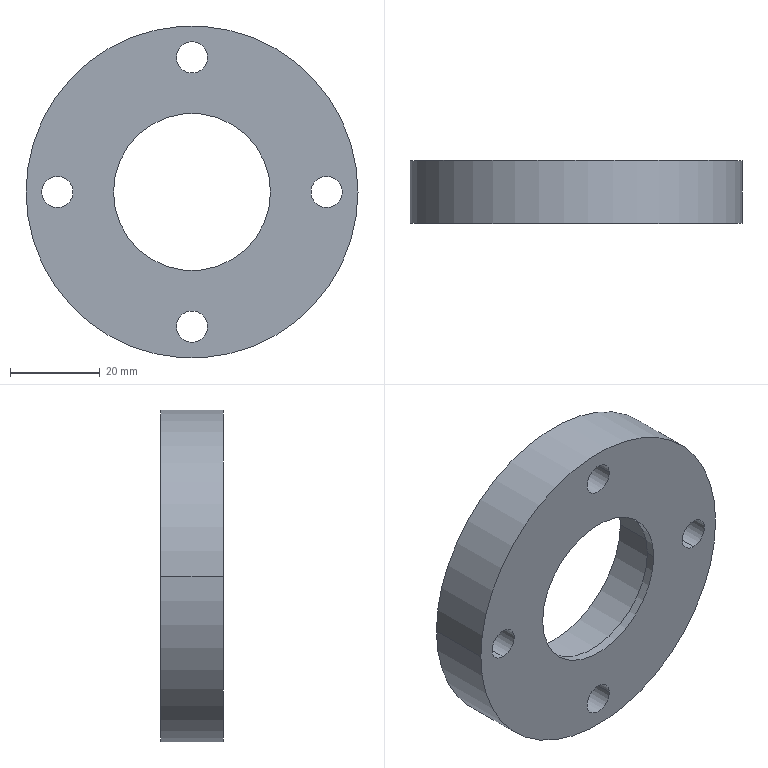Component | SolidWorks | -6004BearingHousing-1 | 1 solid | 29 faces | box 74 x 14 x 74 mm | volume 38150 mm3 | cylinder 22 | plane 7 | commonest cylinder face diameters 11 x8 7 x8 74 x2 42 x2 35 x2
build123d program:
from build123d import *

# Parameters (mm, degrees)
CYLINDRICAL_COUNTERSUNK_HOLE_FOR_M6_HEX_D           = 7
CYLINDRICAL_COUNTERSUNK_HOLE_FOR_M6_HEX_CBORE_D     = 11
CYLINDRICAL_COUNTERSUNK_HOLE_FOR_M6_HEX_CBORE_DEPTH = 6
CIRPATTERN1_COUNT                                   = 4


with BuildPart() as part:
    # Sketch1 → Revolve1 (revolve)
    with BuildSketch(Plane.XY):
        Polygon((17.5, 0), (17.5, 2), (21, 2), (21, 14), (37, 14), (37, 0), align=None)
    revolve(axis=Axis((0, -515.921, 0), (0, 1, 0)))

    # Cylindrical Countersunk Hole for M6 Hex (through all)
    with Locations(Plane(origin=(0, 14, 0), x_dir=(1, 0, 0), z_dir=(0, 1, 0))):
        with Locations((-30, 0)):
            cylindrical_countersunk_hole_for_m6_hex = CounterBoreHole(CYLINDRICAL_COUNTERSUNK_HOLE_FOR_M6_HEX_D / 2, CYLINDRICAL_COUNTERSUNK_HOLE_FOR_M6_HEX_CBORE_D / 2, CYLINDRICAL_COUNTERSUNK_HOLE_FOR_M6_HEX_CBORE_DEPTH)

    # CirPattern1: Cylindrical Countersunk Hole for M6 Hex ×4 about axis
    cirpattern1_axis = Axis((0, 0, 0), (0, 1, 0))
    for i in range(1, CIRPATTERN1_COUNT):
        add(cylindrical_countersunk_hole_for_m6_hex.rotate(cirpattern1_axis, i * 360 / CIRPATTERN1_COUNT), mode=Mode.SUBTRACT)


solid = part.part

# Placed as in the assembly
solid = solid.moved(Location((205, 1451, -173), (0, 0, 0)))
STEP:
#1=CARTESIAN_POINT('',(7.854,57.441,-5.63));
#2=VERTEX_POINT('',#1);
#3=CARTESIAN_POINT('',(8.287,57.441,-5.63));
#4=VERTEX_POINT('',#3);
#5=CARTESIAN_POINT('',(8.071,57.441,-5.63));
#6=DIRECTION('',(-0.,1.,-0.));
#7=DIRECTION('',(1.,0.,0.));
#8=AXIS2_PLACEMENT_3D('',#5,#6,#7);
#9=CIRCLE('',#8,0.2165);
#10=EDGE_CURVE('',#2,#4,#9,.T.);
#11=ORIENTED_EDGE('',*,*,#10,.F.);
#12=CARTESIAN_POINT('',(7.854,57.677,-5.63));
#13=VERTEX_POINT('',#12);
#14=CARTESIAN_POINT('',(7.854,57.677,-5.63));
#15=DIRECTION('',(-0.,1.,-0.));
#16=VECTOR('',#15,39.37);
#17=LINE('',#14,#16);
#18=EDGE_CURVE('',#2,#13,#17,.T.);
#19=ORIENTED_EDGE('',*,*,#18,.T.);
#20=CARTESIAN_POINT('',(8.287,57.677,-5.63));
#21=VERTEX_POINT('',#20);
#22=CARTESIAN_POINT('',(8.071,57.677,-5.63));
#23=DIRECTION('',(-0.,1.,-0.));
#24=DIRECTION('',(1.,0.,0.));
#25=AXIS2_PLACEMENT_3D('',#22,#23,#24);
#26=CIRCLE('',#25,0.2165);
#27=EDGE_CURVE('',#13,#21,#26,.T.);
#28=ORIENTED_EDGE('',*,*,#27,.T.);
#29=CARTESIAN_POINT('',(8.287,57.677,-5.63));
#30=DIRECTION('',(-0.,1.,-0.));
#31=VECTOR('',#30,39.37);
#32=LINE('',#29,#31);
#33=EDGE_CURVE('',#4,#21,#32,.T.);
#34=ORIENTED_EDGE('',*,*,#33,.F.);
#35=EDGE_LOOP('',(#11,#19,#28,#34));
#36=FACE_OUTER_BOUND('',#35,.T.);
#37=CARTESIAN_POINT('',(8.071,57.677,-5.63));
#38=DIRECTION('',(-0.,1.,-0.));
#39=DIRECTION('',(1.,0.,0.));
#40=AXIS2_PLACEMENT_3D('',#37,#38,#39);
#41=CYLINDRICAL_SURFACE('',#40,0.2165);
#42=ADVANCED_FACE('',(#36),#41,.F.);
#43=CARTESIAN_POINT('',(7.933,57.126,-5.63));
#44=VERTEX_POINT('',#43);
#45=CARTESIAN_POINT('',(8.209,57.126,-5.63));
#46=VERTEX_POINT('',#45);
#47=CARTESIAN_POINT('',(8.071,57.126,-5.63));
#48=DIRECTION('',(-0.,1.,-0.));
#49=DIRECTION('',(1.,0.,0.));
#50=AXIS2_PLACEMENT_3D('',#47,#48,#49);
#51=CIRCLE('',#50,0.1378);
#52=EDGE_CURVE('',#44,#46,#51,.T.);
#53=ORIENTED_EDGE('',*,*,#52,.F.);
#54=CARTESIAN_POINT('',(7.933,57.441,-5.63));
#55=VERTEX_POINT('',#54);
#56=CARTESIAN_POINT('',(7.933,57.677,-5.63));
#57=DIRECTION('',(-0.,1.,-0.));
#58=VECTOR('',#57,39.37);
#59=LINE('',#56,#58);
#60=EDGE_CURVE('',#44,#55,#59,.T.);
#61=ORIENTED_EDGE('',*,*,#60,.T.);
#62=CARTESIAN_POINT('',(8.209,57.441,-5.63));
#63=VERTEX_POINT('',#62);
#64=CARTESIAN_POINT('',(8.071,57.441,-5.63));
#65=DIRECTION('',(-0.,1.,-0.));
#66=DIRECTION('',(1.,0.,0.));
#67=AXIS2_PLACEMENT_3D('',#64,#65,#66);
#68=CIRCLE('',#67,0.1378);
#69=EDGE_CURVE('',#55,#63,#68,.T.);
#70=ORIENTED_EDGE('',*,*,#69,.T.);
#71=CARTESIAN_POINT('',(8.209,57.677,-5.63));
#72=DIRECTION('',(-0.,1.,-0.));
#73=VECTOR('',#72,39.37);
#74=LINE('',#71,#73);
#75=EDGE_CURVE('',#46,#63,#74,.T.);
#76=ORIENTED_EDGE('',*,*,#75,.F.);
#77=EDGE_LOOP('',(#53,#61,#70,#76));
#78=FACE_OUTER_BOUND('',#77,.T.);
#79=CARTESIAN_POINT('',(8.071,57.677,-5.63));
#80=DIRECTION('',(-0.,1.,-0.));
#81=DIRECTION('',(1.,0.,0.));
#82=AXIS2_PLACEMENT_3D('',#79,#80,#81);
#83=CYLINDRICAL_SURFACE('',#82,0.1378);
#84=ADVANCED_FACE('',(#78),#83,.F.);
#85=CARTESIAN_POINT('',(9.252,57.441,-6.594));
#86=VERTEX_POINT('',#85);
#87=CARTESIAN_POINT('',(9.252,57.441,-7.028));
#88=VERTEX_POINT('',#87);
#89=CARTESIAN_POINT('',(9.252,57.441,-6.811));
#90=DIRECTION('',(-0.,1.,0.));
#91=DIRECTION('',(0.,0.,-1.));
#92=AXIS2_PLACEMENT_3D('',#89,#90,#91);
#93=CIRCLE('',#92,0.2165);
#94=EDGE_CURVE('',#86,#88,#93,.T.);
#95=ORIENTED_EDGE('',*,*,#94,.F.);
#96=CARTESIAN_POINT('',(9.252,57.677,-6.594));
#97=VERTEX_POINT('',#96);
#98=CARTESIAN_POINT('',(9.252,57.677,-6.594));
#99=DIRECTION('',(-0.,1.,0.));
#100=VECTOR('',#99,39.37);
#101=LINE('',#98,#100);
#102=EDGE_CURVE('',#86,#97,#101,.T.);
#103=ORIENTED_EDGE('',*,*,#102,.T.);
#104=CARTESIAN_POINT('',(9.252,57.677,-7.028));
#105=VERTEX_POINT('',#104);
#106=CARTESIAN_POINT('',(9.252,57.677,-6.811));
#107=DIRECTION('',(-0.,1.,0.));
#108=DIRECTION('',(0.,0.,-1.));
#109=AXIS2_PLACEMENT_3D('',#106,#107,#108);
#110=CIRCLE('',#109,0.2165);
#111=EDGE_CURVE('',#97,#105,#110,.T.);
#112=ORIENTED_EDGE('',*,*,#111,.T.);
#113=CARTESIAN_POINT('',(9.252,57.677,-7.028));
#114=DIRECTION('',(-0.,1.,0.));
#115=VECTOR('',#114,39.37);
#116=LINE('',#113,#115);
#117=EDGE_CURVE('',#88,#105,#116,.T.);
#118=ORIENTED_EDGE('',*,*,#117,.F.);
#119=EDGE_LOOP('',(#95,#103,#112,#118));
#120=FACE_OUTER_BOUND('',#119,.T.);
#121=CARTESIAN_POINT('',(9.252,57.677,-6.811));
#122=DIRECTION('',(-0.,1.,0.));
#123=DIRECTION('',(0.,0.,-1.));
#124=AXIS2_PLACEMENT_3D('',#121,#122,#123);
#125=CYLINDRICAL_SURFACE('',#124,0.2165);
#126=ADVANCED_FACE('',(#120),#125,.F.);
#127=CARTESIAN_POINT('',(9.252,57.126,-6.673));
#128=VERTEX_POINT('',#127);
#129=CARTESIAN_POINT('',(9.252,57.126,-6.949));
#130=VERTEX_POINT('',#129);
#131=CARTESIAN_POINT('',(9.252,57.126,-6.811));
#132=DIRECTION('',(-0.,1.,0.));
#133=DIRECTION('',(0.,0.,-1.));
#134=AXIS2_PLACEMENT_3D('',#131,#132,#133);
#135=CIRCLE('',#134,0.1378);
#136=EDGE_CURVE('',#128,#130,#135,.T.);
#137=ORIENTED_EDGE('',*,*,#136,.F.);
#138=CARTESIAN_POINT('',(9.252,57.441,-6.673));
#139=VERTEX_POINT('',#138);
#140=CARTESIAN_POINT('',(9.252,57.677,-6.673));
#141=DIRECTION('',(-0.,1.,0.));
#142=VECTOR('',#141,39.37);
#143=LINE('',#140,#142);
#144=EDGE_CURVE('',#128,#139,#143,.T.);
#145=ORIENTED_EDGE('',*,*,#144,.T.);
#146=CARTESIAN_POINT('',(9.252,57.441,-6.949));
#147=VERTEX_POINT('',#146);
#148=CARTESIAN_POINT('',(9.252,57.441,-6.811));
#149=DIRECTION('',(-0.,1.,0.));
#150=DIRECTION('',(0.,0.,-1.));
#151=AXIS2_PLACEMENT_3D('',#148,#149,#150);
#152=CIRCLE('',#151,0.1378);
#153=EDGE_CURVE('',#139,#147,#152,.T.);
#154=ORIENTED_EDGE('',*,*,#153,.T.);
#155=CARTESIAN_POINT('',(9.252,57.677,-6.949));
#156=DIRECTION('',(-0.,1.,0.));
#157=VECTOR('',#156,39.37);
#158=LINE('',#155,#157);
#159=EDGE_CURVE('',#130,#147,#158,.T.);
#160=ORIENTED_EDGE('',*,*,#159,.F.);
#161=EDGE_LOOP('',(#137,#145,#154,#160));
#162=FACE_OUTER_BOUND('',#161,.T.);
#163=CARTESIAN_POINT('',(9.252,57.677,-6.811));
#164=DIRECTION('',(-0.,1.,0.));
#165=DIRECTION('',(0.,0.,-1.));
#166=AXIS2_PLACEMENT_3D('',#163,#164,#165);
#167=CYLINDRICAL_SURFACE('',#166,0.1378);
#168=ADVANCED_FACE('',(#162),#167,.F.);
#169=CARTESIAN_POINT('',(8.287,57.441,-7.992));
#170=VERTEX_POINT('',#169);
#171=CARTESIAN_POINT('',(7.854,57.441,-7.992));
#172=VERTEX_POINT('',#171);
#173=CARTESIAN_POINT('',(8.071,57.441,-7.992));
#174=DIRECTION('',(-0.,1.,0.));
#175=DIRECTION('',(-1.,0.,-0.));
#176=AXIS2_PLACEMENT_3D('',#173,#174,#175);
#177=CIRCLE('',#176,0.2165);
#178=EDGE_CURVE('',#170,#172,#177,.T.);
#179=ORIENTED_EDGE('',*,*,#178,.F.);
#180=CARTESIAN_POINT('',(8.287,57.677,-7.992));
#181=VERTEX_POINT('',#180);
#182=CARTESIAN_POINT('',(8.287,57.677,-7.992));
#183=DIRECTION('',(-0.,1.,0.));
#184=VECTOR('',#183,39.37);
#185=LINE('',#182,#184);
#186=EDGE_CURVE('',#170,#181,#185,.T.);
#187=ORIENTED_EDGE('',*,*,#186,.T.);
#188=CARTESIAN_POINT('',(7.854,57.677,-7.992));
#189=VERTEX_POINT('',#188);
#190=CARTESIAN_POINT('',(8.071,57.677,-7.992));
#191=DIRECTION('',(-0.,1.,0.));
#192=DIRECTION('',(-1.,0.,-0.));
#193=AXIS2_PLACEMENT_3D('',#190,#191,#192);
#194=CIRCLE('',#193,0.2165);
#195=EDGE_CURVE('',#181,#189,#194,.T.);
#196=ORIENTED_EDGE('',*,*,#195,.T.);
#197=CARTESIAN_POINT('',(7.854,57.677,-7.992));
#198=DIRECTION('',(-0.,1.,0.));
#199=VECTOR('',#198,39.37);
#200=LINE('',#197,#199);
#201=EDGE_CURVE('',#172,#189,#200,.T.);
#202=ORIENTED_EDGE('',*,*,#201,.F.);
#203=EDGE_LOOP('',(#179,#187,#196,#202));
#204=FACE_OUTER_BOUND('',#203,.T.);
#205=CARTESIAN_POINT('',(8.071,57.677,-7.992));
#206=DIRECTION('',(-0.,1.,0.));
#207=DIRECTION('',(-1.,0.,-0.));
#208=AXIS2_PLACEMENT_3D('',#205,#206,#207);
#209=CYLINDRICAL_SURFACE('',#208,0.2165);
#210=ADVANCED_FACE('',(#204),#209,.F.);
#211=CARTESIAN_POINT('',(8.209,57.126,-7.992));
#212=VERTEX_POINT('',#211);
#213=CARTESIAN_POINT('',(7.933,57.126,-7.992));
#214=VERTEX_POINT('',#213);
#215=CARTESIAN_POINT('',(8.071,57.126,-7.992));
#216=DIRECTION('',(-0.,1.,0.));
#217=DIRECTION('',(-1.,0.,0.));
#218=AXIS2_PLACEMENT_3D('',#215,#216,#217);
#219=CIRCLE('',#218,0.1378);
#220=EDGE_CURVE('',#212,#214,#219,.T.);
#221=ORIENTED_EDGE('',*,*,#220,.F.);
#222=CARTESIAN_POINT('',(8.209,57.441,-7.992));
#223=VERTEX_POINT('',#222);
#224=CARTESIAN_POINT('',(8.209,57.677,-7.992));
#225=DIRECTION('',(-0.,1.,0.));
#226=VECTOR('',#225,39.37);
#227=LINE('',#224,#226);
#228=EDGE_CURVE('',#212,#223,#227,.T.);
#229=ORIENTED_EDGE('',*,*,#228,.T.);
#230=CARTESIAN_POINT('',(7.933,57.441,-7.992));
#231=VERTEX_POINT('',#230);
#232=CARTESIAN_POINT('',(8.071,57.441,-7.992));
#233=DIRECTION('',(-0.,1.,0.));
#234=DIRECTION('',(-1.,0.,0.));
#235=AXIS2_PLACEMENT_3D('',#232,#233,#234);
#236=CIRCLE('',#235,0.1378);
#237=EDGE_CURVE('',#223,#231,#236,.T.);
#238=ORIENTED_EDGE('',*,*,#237,.T.);
#239=CARTESIAN_POINT('',(7.933,57.677,-7.992));
#240=DIRECTION('',(-0.,1.,0.));
#241=VECTOR('',#240,39.37);
#242=LINE('',#239,#241);
#243=EDGE_CURVE('',#214,#231,#242,.T.);
#244=ORIENTED_EDGE('',*,*,#243,.F.);
#245=EDGE_LOOP('',(#221,#229,#238,#244));
#246=FACE_OUTER_BOUND('',#245,.T.);
#247=CARTESIAN_POINT('',(8.071,57.677,-7.992));
#248=DIRECTION('',(-0.,1.,0.));
#249=DIRECTION('',(-1.,0.,0.));
#250=AXIS2_PLACEMENT_3D('',#247,#248,#249);
#251=CYLINDRICAL_SURFACE('',#250,0.1378);
#252=ADVANCED_FACE('',(#246),#251,.F.);
#253=CARTESIAN_POINT('',(6.89,57.441,-7.028));
#254=VERTEX_POINT('',#253);
#255=CARTESIAN_POINT('',(6.89,57.441,-6.594));
#256=VERTEX_POINT('',#255);
#257=CARTESIAN_POINT('',(6.89,57.441,-6.811));
#258=DIRECTION('',(0.,1.,0.));
#259=DIRECTION('',(0.,0.,1.));
#260=AXIS2_PLACEMENT_3D('',#257,#258,#259);
#261=CIRCLE('',#260,0.2165);
#262=EDGE_CURVE('',#254,#256,#261,.T.);
#263=ORIENTED_EDGE('',*,*,#262,.F.);
#264=CARTESIAN_POINT('',(6.89,57.677,-7.028));
#265=VERTEX_POINT('',#264);
#266=CARTESIAN_POINT('',(6.89,57.677,-7.028));
#267=DIRECTION('',(0.,1.,0.));
#268=VECTOR('',#267,39.37);
#269=LINE('',#266,#268);
#270=EDGE_CURVE('',#254,#265,#269,.T.);
#271=ORIENTED_EDGE('',*,*,#270,.T.);
#272=CARTESIAN_POINT('',(6.89,57.677,-6.594));
#273=VERTEX_POINT('',#272);
#274=CARTESIAN_POINT('',(6.89,57.677,-6.811));
#275=DIRECTION('',(0.,1.,0.));
#276=DIRECTION('',(0.,0.,1.));
#277=AXIS2_PLACEMENT_3D('',#274,#275,#276);
#278=CIRCLE('',#277,0.2165);
#279=EDGE_CURVE('',#265,#273,#278,.T.);
#280=ORIENTED_EDGE('',*,*,#279,.T.);
#281=CARTESIAN_POINT('',(6.89,57.677,-6.594));
#282=DIRECTION('',(0.,1.,0.));
#283=VECTOR('',#282,39.37);
#284=LINE('',#281,#283);
#285=EDGE_CURVE('',#256,#273,#284,.T.);
#286=ORIENTED_EDGE('',*,*,#285,.F.);
#287=EDGE_LOOP('',(#263,#271,#280,#286));
#288=FACE_OUTER_BOUND('',#287,.T.);
#289=CARTESIAN_POINT('',(6.89,57.677,-6.811));
#290=DIRECTION('',(0.,1.,0.));
#291=DIRECTION('',(0.,0.,1.));
#292=AXIS2_PLACEMENT_3D('',#289,#290,#291);
#293=CYLINDRICAL_SURFACE('',#292,0.2165);
#294=ADVANCED_FACE('',(#288),#293,.F.);
#295=CARTESIAN_POINT('',(6.89,57.126,-6.949));
#296=VERTEX_POINT('',#295);
#297=CARTESIAN_POINT('',(6.89,57.126,-6.673));
#298=VERTEX_POINT('',#297);
#299=CARTESIAN_POINT('',(6.89,57.126,-6.811));
#300=DIRECTION('',(0.,1.,0.));
#301=DIRECTION('',(0.,0.,1.));
#302=AXIS2_PLACEMENT_3D('',#299,#300,#301);
#303=CIRCLE('',#302,0.1378);
#304=EDGE_CURVE('',#296,#298,#303,.T.);
#305=ORIENTED_EDGE('',*,*,#304,.F.);
#306=CARTESIAN_POINT('',(6.89,57.441,-6.949));
#307=VERTEX_POINT('',#306);
#308=CARTESIAN_POINT('',(6.89,57.677,-6.949));
#309=DIRECTION('',(0.,1.,0.));
#310=VECTOR('',#309,39.37);
#311=LINE('',#308,#310);
#312=EDGE_CURVE('',#296,#307,#311,.T.);
#313=ORIENTED_EDGE('',*,*,#312,.T.);
#314=CARTESIAN_POINT('',(6.89,57.441,-6.673));
#315=VERTEX_POINT('',#314);
#316=CARTESIAN_POINT('',(6.89,57.441,-6.811));
#317=DIRECTION('',(0.,1.,0.));
#318=DIRECTION('',(0.,0.,1.));
#319=AXIS2_PLACEMENT_3D('',#316,#317,#318);
#320=CIRCLE('',#319,0.1378);
#321=EDGE_CURVE('',#307,#315,#320,.T.);
#322=ORIENTED_EDGE('',*,*,#321,.T.);
#323=CARTESIAN_POINT('',(6.89,57.677,-6.673));
#324=DIRECTION('',(0.,1.,0.));
#325=VECTOR('',#324,39.37);
#326=LINE('',#323,#325);
#327=EDGE_CURVE('',#298,#315,#326,.T.);
#328=ORIENTED_EDGE('',*,*,#327,.F.);
#329=EDGE_LOOP('',(#305,#313,#322,#328));
#330=FACE_OUTER_BOUND('',#329,.T.);
#331=CARTESIAN_POINT('',(6.89,57.677,-6.811));
#332=DIRECTION('',(0.,1.,0.));
#333=DIRECTION('',(0.,0.,1.));
#334=AXIS2_PLACEMENT_3D('',#331,#332,#333);
#335=CYLINDRICAL_SURFACE('',#334,0.1378);
#336=ADVANCED_FACE('',(#330),#335,.F.);
#337=CARTESIAN_POINT('',(9.528,57.677,-6.811));
#338=VERTEX_POINT('',#337);
#339=CARTESIAN_POINT('',(6.614,57.677,-6.811));
#340=VERTEX_POINT('',#339);
#341=CARTESIAN_POINT('',(8.071,57.677,-6.811));
#342=DIRECTION('',(0.,-1.,0.));
#343=DIRECTION('',(1.,0.,0.));
#344=AXIS2_PLACEMENT_3D('',#341,#342,#343);
#345=CIRCLE('',#344,1.457);
#346=EDGE_CURVE('',#338,#340,#345,.T.);
#347=ORIENTED_EDGE('',*,*,#346,.T.);
#348=CARTESIAN_POINT('',(6.614,57.126,-6.811));
#349=VERTEX_POINT('',#348);
#350=CARTESIAN_POINT('',(6.614,36.814,-6.811));
#351=DIRECTION('',(0.,-1.,0.));
#352=VECTOR('',#351,39.37);
#353=LINE('',#350,#352);
#354=EDGE_CURVE('',#340,#349,#353,.T.);
#355=ORIENTED_EDGE('',*,*,#354,.T.);
#356=CARTESIAN_POINT('',(9.528,57.126,-6.811));
#357=VERTEX_POINT('',#356);
#358=CARTESIAN_POINT('',(8.071,57.126,-6.811));
#359=DIRECTION('',(0.,-1.,0.));
#360=DIRECTION('',(1.,0.,0.));
#361=AXIS2_PLACEMENT_3D('',#358,#359,#360);
#362=CIRCLE('',#361,1.457);
#363=EDGE_CURVE('',#357,#349,#362,.T.);
#364=ORIENTED_EDGE('',*,*,#363,.F.);
#365=CARTESIAN_POINT('',(9.528,36.814,-6.811));
#366=DIRECTION('',(0.,-1.,0.));
#367=VECTOR('',#366,39.37);
#368=LINE('',#365,#367);
#369=EDGE_CURVE('',#338,#357,#368,.T.);
#370=ORIENTED_EDGE('',*,*,#369,.F.);
#371=EDGE_LOOP('',(#347,#355,#364,#370));
#372=FACE_OUTER_BOUND('',#371,.T.);
#373=CARTESIAN_POINT('',(8.071,36.814,-6.811));
#374=DIRECTION('',(0.,-1.,0.));
#375=DIRECTION('',(1.,0.,0.));
#376=AXIS2_PLACEMENT_3D('',#373,#374,#375);
#377=CYLINDRICAL_SURFACE('',#376,1.457);
#378=ADVANCED_FACE('',(#372),#377,.T.);
#379=CARTESIAN_POINT('',(7.244,57.677,-6.811));
#380=VERTEX_POINT('',#379);
#381=CARTESIAN_POINT('',(8.898,57.677,-6.811));
#382=VERTEX_POINT('',#381);
#383=CARTESIAN_POINT('',(8.071,57.677,-6.811));
#384=DIRECTION('',(0.,-1.,0.));
#385=DIRECTION('',(1.,0.,0.));
#386=AXIS2_PLACEMENT_3D('',#383,#384,#385);
#387=CIRCLE('',#386,0.8268);
#388=EDGE_CURVE('',#380,#382,#387,.T.);
#389=ORIENTED_EDGE('',*,*,#388,.F.);
#390=CARTESIAN_POINT('',(7.244,57.205,-6.811));
#391=VERTEX_POINT('',#390);
#392=CARTESIAN_POINT('',(7.244,36.814,-6.811));
#393=DIRECTION('',(0.,-1.,0.));
#394=VECTOR('',#393,39.37);
#395=LINE('',#392,#394);
#396=EDGE_CURVE('',#380,#391,#395,.T.);
#397=ORIENTED_EDGE('',*,*,#396,.T.);
#398=CARTESIAN_POINT('',(8.898,57.205,-6.811));
#399=VERTEX_POINT('',#398);
#400=CARTESIAN_POINT('',(8.071,57.205,-6.811));
#401=DIRECTION('',(0.,-1.,0.));
#402=DIRECTION('',(1.,0.,0.));
#403=AXIS2_PLACEMENT_3D('',#400,#401,#402);
#404=CIRCLE('',#403,0.8268);
#405=EDGE_CURVE('',#391,#399,#404,.T.);
#406=ORIENTED_EDGE('',*,*,#405,.T.);
#407=CARTESIAN_POINT('',(8.898,36.814,-6.811));
#408=DIRECTION('',(0.,-1.,0.));
#409=VECTOR('',#408,39.37);
#410=LINE('',#407,#409);
#411=EDGE_CURVE('',#382,#399,#410,.T.);
#412=ORIENTED_EDGE('',*,*,#411,.F.);
#413=EDGE_LOOP('',(#389,#397,#406,#412));
#414=FACE_OUTER_BOUND('',#413,.T.);
#415=CARTESIAN_POINT('',(8.071,36.814,-6.811));
#416=DIRECTION('',(0.,-1.,0.));
#417=DIRECTION('',(1.,0.,0.));
#418=AXIS2_PLACEMENT_3D('',#415,#416,#417);
#419=CYLINDRICAL_SURFACE('',#418,0.8268);
#420=ADVANCED_FACE('',(#414),#419,.F.);
#421=CARTESIAN_POINT('',(7.382,57.205,-6.811));
#422=VERTEX_POINT('',#421);
#423=CARTESIAN_POINT('',(8.76,57.205,-6.811));
#424=VERTEX_POINT('',#423);
#425=CARTESIAN_POINT('',(8.071,57.205,-6.811));
#426=DIRECTION('',(0.,-1.,0.));
#427=DIRECTION('',(1.,0.,0.));
#428=AXIS2_PLACEMENT_3D('',#425,#426,#427);
#429=CIRCLE('',#428,0.689);
#430=EDGE_CURVE('',#422,#424,#429,.T.);
#431=ORIENTED_EDGE('',*,*,#430,.F.);
#432=CARTESIAN_POINT('',(7.382,57.126,-6.811));
#433=VERTEX_POINT('',#432);
#434=CARTESIAN_POINT('',(7.382,36.814,-6.811));
#435=DIRECTION('',(0.,-1.,0.));
#436=VECTOR('',#435,39.37);
#437=LINE('',#434,#436);
#438=EDGE_CURVE('',#422,#433,#437,.T.);
#439=ORIENTED_EDGE('',*,*,#438,.T.);
#440=CARTESIAN_POINT('',(8.76,57.126,-6.811));
#441=VERTEX_POINT('',#440);
#442=CARTESIAN_POINT('',(8.071,57.126,-6.811));
#443=DIRECTION('',(0.,-1.,0.));
#444=DIRECTION('',(1.,0.,0.));
#445=AXIS2_PLACEMENT_3D('',#442,#443,#444);
#446=CIRCLE('',#445,0.689);
#447=EDGE_CURVE('',#433,#441,#446,.T.);
#448=ORIENTED_EDGE('',*,*,#447,.T.);
#449=CARTESIAN_POINT('',(8.76,36.814,-6.811));
#450=DIRECTION('',(0.,-1.,0.));
#451=VECTOR('',#450,39.37);
#452=LINE('',#449,#451);
#453=EDGE_CURVE('',#424,#441,#452,.T.);
#454=ORIENTED_EDGE('',*,*,#453,.F.);
#455=EDGE_LOOP('',(#431,#439,#448,#454));
#456=FACE_OUTER_BOUND('',#455,.T.);
#457=CARTESIAN_POINT('',(8.071,36.814,-6.811));
#458=DIRECTION('',(0.,-1.,0.));
#459=DIRECTION('',(1.,0.,0.));
#460=AXIS2_PLACEMENT_3D('',#457,#458,#459);
#461=CYLINDRICAL_SURFACE('',#460,0.689);
#462=ADVANCED_FACE('',(#456),#461,.F.);
#463=CARTESIAN_POINT('',(8.071,57.126,-5.63));
#464=DIRECTION('',(-0.,1.,-0.));
#465=DIRECTION('',(1.,0.,0.));
#466=AXIS2_PLACEMENT_3D('',#463,#464,#465);
#467=CIRCLE('',#466,0.1378);
#468=EDGE_CURVE('',#46,#44,#467,.T.);
#469=ORIENTED_EDGE('',*,*,#468,.T.);
#470=ORIENTED_EDGE('',*,*,#52,.T.);
#471=EDGE_LOOP('',(#469,#470));
#472=FACE_BOUND('',#471,.T.);
#473=CARTESIAN_POINT('',(9.252,57.126,-6.811));
#474=DIRECTION('',(-0.,1.,0.));
#475=DIRECTION('',(0.,0.,-1.));
#476=AXIS2_PLACEMENT_3D('',#473,#474,#475);
#477=CIRCLE('',#476,0.1378);
#478=EDGE_CURVE('',#130,#128,#477,.T.);
#479=ORIENTED_EDGE('',*,*,#478,.T.);
#480=ORIENTED_EDGE('',*,*,#136,.T.);
#481=EDGE_LOOP('',(#479,#480));
#482=FACE_BOUND('',#481,.T.);
#483=CARTESIAN_POINT('',(8.071,57.126,-7.992));
#484=DIRECTION('',(-0.,1.,0.));
#485=DIRECTION('',(-1.,0.,0.));
#486=AXIS2_PLACEMENT_3D('',#483,#484,#485);
#487=CIRCLE('',#486,0.1378);
#488=EDGE_CURVE('',#214,#212,#487,.T.);
#489=ORIENTED_EDGE('',*,*,#488,.T.);
#490=ORIENTED_EDGE('',*,*,#220,.T.);
#491=EDGE_LOOP('',(#489,#490));
#492=FACE_BOUND('',#491,.T.);
#493=CARTESIAN_POINT('',(6.89,57.126,-6.811));
#494=DIRECTION('',(0.,1.,0.));
#495=DIRECTION('',(0.,0.,1.));
#496=AXIS2_PLACEMENT_3D('',#493,#494,#495);
#497=CIRCLE('',#496,0.1378);
#498=EDGE_CURVE('',#298,#296,#497,.T.);
#499=ORIENTED_EDGE('',*,*,#498,.T.);
#500=ORIENTED_EDGE('',*,*,#304,.T.);
#501=EDGE_LOOP('',(#499,#500));
#502=FACE_BOUND('',#501,.T.);
#503=ORIENTED_EDGE('',*,*,#363,.T.);
#504=CARTESIAN_POINT('',(8.071,57.126,-6.811));
#505=DIRECTION('',(0.,-1.,0.));
#506=DIRECTION('',(1.,0.,0.));
#507=AXIS2_PLACEMENT_3D('',#504,#505,#506);
#508=CIRCLE('',#507,1.457);
#509=EDGE_CURVE('',#349,#357,#508,.T.);
#510=ORIENTED_EDGE('',*,*,#509,.T.);
#511=EDGE_LOOP('',(#503,#510));
#512=FACE_OUTER_BOUND('',#511,.T.);
#513=CARTESIAN_POINT('',(8.071,57.126,-6.811));
#514=DIRECTION('',(0.,-1.,0.));
#515=DIRECTION('',(1.,0.,0.));
#516=AXIS2_PLACEMENT_3D('',#513,#514,#515);
#517=CIRCLE('',#516,0.689);
#518=EDGE_CURVE('',#441,#433,#517,.T.);
#519=ORIENTED_EDGE('',*,*,#518,.F.);
#520=ORIENTED_EDGE('',*,*,#447,.F.);
#521=EDGE_LOOP('',(#519,#520));
#522=FACE_BOUND('',#521,.T.);
#523=CARTESIAN_POINT('',(9.528,57.126,-6.811));
#524=DIRECTION('',(0.,-1.,0.));
#525=DIRECTION('',(1.,0.,0.));
#526=AXIS2_PLACEMENT_3D('',#523,#524,#525);
#527=PLANE('',#526);
#528=ADVANCED_FACE('',(#472,#482,#492,#502,#512,#522),#527,.T.);
#529=ORIENTED_EDGE('',*,*,#438,.F.);
#530=CARTESIAN_POINT('',(8.071,57.205,-6.811));
#531=DIRECTION('',(0.,-1.,0.));
#532=DIRECTION('',(1.,0.,0.));
#533=AXIS2_PLACEMENT_3D('',#530,#531,#532);
#534=CIRCLE('',#533,0.689);
#535=EDGE_CURVE('',#424,#422,#534,.T.);
#536=ORIENTED_EDGE('',*,*,#535,.F.);
#537=ORIENTED_EDGE('',*,*,#453,.T.);
#538=ORIENTED_EDGE('',*,*,#518,.T.);
#539=EDGE_LOOP('',(#529,#536,#537,#538));
#540=FACE_OUTER_BOUND('',#539,.T.);
#541=CARTESIAN_POINT('',(8.071,36.814,-6.811));
#542=DIRECTION('',(0.,-1.,0.));
#543=DIRECTION('',(1.,0.,0.));
#544=AXIS2_PLACEMENT_3D('',#541,#542,#543);
#545=CYLINDRICAL_SURFACE('',#544,0.689);
#546=ADVANCED_FACE('',(#540),#545,.F.);
#547=ORIENTED_EDGE('',*,*,#535,.T.);
#548=ORIENTED_EDGE('',*,*,#430,.T.);
#549=EDGE_LOOP('',(#547,#548));
#550=FACE_BOUND('',#549,.T.);
#551=CARTESIAN_POINT('',(8.071,57.205,-6.811));
#552=DIRECTION('',(0.,-1.,0.));
#553=DIRECTION('',(1.,0.,0.));
#554=AXIS2_PLACEMENT_3D('',#551,#552,#553);
#555=CIRCLE('',#554,0.8268);
#556=EDGE_CURVE('',#399,#391,#555,.T.);
#557=ORIENTED_EDGE('',*,*,#556,.F.);
#558=ORIENTED_EDGE('',*,*,#405,.F.);
#559=EDGE_LOOP('',(#557,#558));
#560=FACE_OUTER_BOUND('',#559,.T.);
#561=CARTESIAN_POINT('',(8.76,57.205,-6.811));
#562=DIRECTION('',(-0.,1.,0.));
#563=DIRECTION('',(-1.,-0.,0.));
#564=AXIS2_PLACEMENT_3D('',#561,#562,#563);
#565=PLANE('',#564);
#566=ADVANCED_FACE('',(#550,#560),#565,.T.);
#567=ORIENTED_EDGE('',*,*,#396,.F.);
#568=CARTESIAN_POINT('',(8.071,57.677,-6.811));
#569=DIRECTION('',(0.,-1.,0.));
#570=DIRECTION('',(1.,0.,0.));
#571=AXIS2_PLACEMENT_3D('',#568,#569,#570);
#572=CIRCLE('',#571,0.8268);
#573=EDGE_CURVE('',#382,#380,#572,.T.);
#574=ORIENTED_EDGE('',*,*,#573,.F.);
#575=ORIENTED_EDGE('',*,*,#411,.T.);
#576=ORIENTED_EDGE('',*,*,#556,.T.);
#577=EDGE_LOOP('',(#567,#574,#575,#576));
#578=FACE_OUTER_BOUND('',#577,.T.);
#579=CARTESIAN_POINT('',(8.071,36.814,-6.811));
#580=DIRECTION('',(0.,-1.,0.));
#581=DIRECTION('',(1.,0.,0.));
#582=AXIS2_PLACEMENT_3D('',#579,#580,#581);
#583=CYLINDRICAL_SURFACE('',#582,0.8268);
#584=ADVANCED_FACE('',(#578),#583,.F.);
#585=CARTESIAN_POINT('',(8.071,57.677,-5.63));
#586=DIRECTION('',(-0.,1.,-0.));
#587=DIRECTION('',(1.,0.,0.));
#588=AXIS2_PLACEMENT_3D('',#585,#586,#587);
#589=CIRCLE('',#588,0.2165);
#590=EDGE_CURVE('',#21,#13,#589,.T.);
#591=ORIENTED_EDGE('',*,*,#590,.F.);
#592=ORIENTED_EDGE('',*,*,#27,.F.);
#593=EDGE_LOOP('',(#591,#592));
#594=FACE_BOUND('',#593,.T.);
#595=CARTESIAN_POINT('',(9.252,57.677,-6.811));
#596=DIRECTION('',(-0.,1.,0.));
#597=DIRECTION('',(0.,0.,-1.));
#598=AXIS2_PLACEMENT_3D('',#595,#596,#597);
#599=CIRCLE('',#598,0.2165);
#600=EDGE_CURVE('',#105,#97,#599,.T.);
#601=ORIENTED_EDGE('',*,*,#600,.F.);
#602=ORIENTED_EDGE('',*,*,#111,.F.);
#603=EDGE_LOOP('',(#601,#602));
#604=FACE_BOUND('',#603,.T.);
#605=CARTESIAN_POINT('',(8.071,57.677,-7.992));
#606=DIRECTION('',(-0.,1.,0.));
#607=DIRECTION('',(-1.,0.,-0.));
#608=AXIS2_PLACEMENT_3D('',#605,#606,#607);
#609=CIRCLE('',#608,0.2165);
#610=EDGE_CURVE('',#189,#181,#609,.T.);
#611=ORIENTED_EDGE('',*,*,#610,.F.);
#612=ORIENTED_EDGE('',*,*,#195,.F.);
#613=EDGE_LOOP('',(#611,#612));
#614=FACE_BOUND('',#613,.T.);
#615=CARTESIAN_POINT('',(6.89,57.677,-6.811));
#616=DIRECTION('',(0.,1.,0.));
#617=DIRECTION('',(0.,0.,1.));
#618=AXIS2_PLACEMENT_3D('',#615,#616,#617);
#619=CIRCLE('',#618,0.2165);
#620=EDGE_CURVE('',#273,#265,#619,.T.);
#621=ORIENTED_EDGE('',*,*,#620,.F.);
#622=ORIENTED_EDGE('',*,*,#279,.F.);
#623=EDGE_LOOP('',(#621,#622));
#624=FACE_BOUND('',#623,.T.);
#625=ORIENTED_EDGE('',*,*,#573,.T.);
#626=ORIENTED_EDGE('',*,*,#388,.T.);
#627=EDGE_LOOP('',(#625,#626));
#628=FACE_BOUND('',#627,.T.);
#629=ORIENTED_EDGE('',*,*,#346,.F.);
#630=CARTESIAN_POINT('',(8.071,57.677,-6.811));
#631=DIRECTION('',(0.,-1.,0.));
#632=DIRECTION('',(1.,0.,0.));
#633=AXIS2_PLACEMENT_3D('',#630,#631,#632);
#634=CIRCLE('',#633,1.457);
#635=EDGE_CURVE('',#340,#338,#634,.T.);
#636=ORIENTED_EDGE('',*,*,#635,.F.);
#637=EDGE_LOOP('',(#629,#636));
#638=FACE_OUTER_BOUND('',#637,.T.);
#639=CARTESIAN_POINT('',(8.898,57.677,-6.811));
#640=DIRECTION('',(-0.,1.,0.));
#641=DIRECTION('',(-1.,-0.,0.));
#642=AXIS2_PLACEMENT_3D('',#639,#640,#641);
#643=PLANE('',#642);
#644=ADVANCED_FACE('',(#594,#604,#614,#624,#628,#638),#643,.T.);
#645=ORIENTED_EDGE('',*,*,#354,.F.);
#646=ORIENTED_EDGE('',*,*,#635,.T.);
#647=ORIENTED_EDGE('',*,*,#369,.T.);
#648=ORIENTED_EDGE('',*,*,#509,.F.);
#649=EDGE_LOOP('',(#645,#646,#647,#648));
#650=FACE_OUTER_BOUND('',#649,.T.);
#651=CARTESIAN_POINT('',(8.071,36.814,-6.811));
#652=DIRECTION('',(0.,-1.,0.));
#653=DIRECTION('',(1.,0.,0.));
#654=AXIS2_PLACEMENT_3D('',#651,#652,#653);
#655=CYLINDRICAL_SURFACE('',#654,1.457);
#656=ADVANCED_FACE('',(#650),#655,.T.);
#657=ORIENTED_EDGE('',*,*,#312,.F.);
#658=ORIENTED_EDGE('',*,*,#498,.F.);
#659=ORIENTED_EDGE('',*,*,#327,.T.);
#660=CARTESIAN_POINT('',(6.89,57.441,-6.811));
#661=DIRECTION('',(0.,1.,0.));
#662=DIRECTION('',(0.,0.,1.));
#663=AXIS2_PLACEMENT_3D('',#660,#661,#662);
#664=CIRCLE('',#663,0.1378);
#665=EDGE_CURVE('',#315,#307,#664,.T.);
#666=ORIENTED_EDGE('',*,*,#665,.T.);
#667=EDGE_LOOP('',(#657,#658,#659,#666));
#668=FACE_OUTER_BOUND('',#667,.T.);
#669=CARTESIAN_POINT('',(6.89,57.677,-6.811));
#670=DIRECTION('',(0.,1.,0.));
#671=DIRECTION('',(0.,0.,1.));
#672=AXIS2_PLACEMENT_3D('',#669,#670,#671);
#673=CYLINDRICAL_SURFACE('',#672,0.1378);
#674=ADVANCED_FACE('',(#668),#673,.F.);
#675=ORIENTED_EDGE('',*,*,#665,.F.);
#676=ORIENTED_EDGE('',*,*,#321,.F.);
#677=EDGE_LOOP('',(#675,#676));
#678=FACE_BOUND('',#677,.T.);
#679=CARTESIAN_POINT('',(6.89,57.441,-6.811));
#680=DIRECTION('',(0.,1.,0.));
#681=DIRECTION('',(0.,0.,1.));
#682=AXIS2_PLACEMENT_3D('',#679,#680,#681);
#683=CIRCLE('',#682,0.2165);
#684=EDGE_CURVE('',#256,#254,#683,.T.);
#685=ORIENTED_EDGE('',*,*,#684,.T.);
#686=ORIENTED_EDGE('',*,*,#262,.T.);
#687=EDGE_LOOP('',(#685,#686));
#688=FACE_OUTER_BOUND('',#687,.T.);
#689=CARTESIAN_POINT('',(7.028,57.441,-6.811));
#690=DIRECTION('',(0.,-1.,0.));
#691=DIRECTION('',(0.,0.,-1.));
#692=AXIS2_PLACEMENT_3D('',#689,#690,#691);
#693=PLANE('',#692);
#694=ADVANCED_FACE('',(#678,#688),#693,.F.);
#695=ORIENTED_EDGE('',*,*,#270,.F.);
#696=ORIENTED_EDGE('',*,*,#684,.F.);
#697=ORIENTED_EDGE('',*,*,#285,.T.);
#698=ORIENTED_EDGE('',*,*,#620,.T.);
#699=EDGE_LOOP('',(#695,#696,#697,#698));
#700=FACE_OUTER_BOUND('',#699,.T.);
#701=CARTESIAN_POINT('',(6.89,57.677,-6.811));
#702=DIRECTION('',(0.,1.,0.));
#703=DIRECTION('',(0.,0.,1.));
#704=AXIS2_PLACEMENT_3D('',#701,#702,#703);
#705=CYLINDRICAL_SURFACE('',#704,0.2165);
#706=ADVANCED_FACE('',(#700),#705,.F.);
#707=ORIENTED_EDGE('',*,*,#228,.F.);
#708=ORIENTED_EDGE('',*,*,#488,.F.);
#709=ORIENTED_EDGE('',*,*,#243,.T.);
#710=CARTESIAN_POINT('',(8.071,57.441,-7.992));
#711=DIRECTION('',(-0.,1.,0.));
#712=DIRECTION('',(-1.,0.,0.));
#713=AXIS2_PLACEMENT_3D('',#710,#711,#712);
#714=CIRCLE('',#713,0.1378);
#715=EDGE_CURVE('',#231,#223,#714,.T.);
#716=ORIENTED_EDGE('',*,*,#715,.T.);
#717=EDGE_LOOP('',(#707,#708,#709,#716));
#718=FACE_OUTER_BOUND('',#717,.T.);
#719=CARTESIAN_POINT('',(8.071,57.677,-7.992));
#720=DIRECTION('',(-0.,1.,0.));
#721=DIRECTION('',(-1.,0.,0.));
#722=AXIS2_PLACEMENT_3D('',#719,#720,#721);
#723=CYLINDRICAL_SURFACE('',#722,0.1378);
#724=ADVANCED_FACE('',(#718),#723,.F.);
#725=ORIENTED_EDGE('',*,*,#715,.F.);
#726=ORIENTED_EDGE('',*,*,#237,.F.);
#727=EDGE_LOOP('',(#725,#726));
#728=FACE_BOUND('',#727,.T.);
#729=CARTESIAN_POINT('',(8.071,57.441,-7.992));
#730=DIRECTION('',(-0.,1.,0.));
#731=DIRECTION('',(-1.,0.,-0.));
#732=AXIS2_PLACEMENT_3D('',#729,#730,#731);
#733=CIRCLE('',#732,0.2165);
#734=EDGE_CURVE('',#172,#170,#733,.T.);
#735=ORIENTED_EDGE('',*,*,#734,.T.);
#736=ORIENTED_EDGE('',*,*,#178,.T.);
#737=EDGE_LOOP('',(#735,#736));
#738=FACE_OUTER_BOUND('',#737,.T.);
#739=CARTESIAN_POINT('',(8.071,57.441,-7.854));
#740=DIRECTION('',(0.,-1.,-0.));
#741=DIRECTION('',(1.,0.,0.));
#742=AXIS2_PLACEMENT_3D('',#739,#740,#741);
#743=PLANE('',#742);
#744=ADVANCED_FACE('',(#728,#738),#743,.F.);
#745=ORIENTED_EDGE('',*,*,#186,.F.);
#746=ORIENTED_EDGE('',*,*,#734,.F.);
#747=ORIENTED_EDGE('',*,*,#201,.T.);
#748=ORIENTED_EDGE('',*,*,#610,.T.);
#749=EDGE_LOOP('',(#745,#746,#747,#748));
#750=FACE_OUTER_BOUND('',#749,.T.);
#751=CARTESIAN_POINT('',(8.071,57.677,-7.992));
#752=DIRECTION('',(-0.,1.,0.));
#753=DIRECTION('',(-1.,0.,-0.));
#754=AXIS2_PLACEMENT_3D('',#751,#752,#753);
#755=CYLINDRICAL_SURFACE('',#754,0.2165);
#756=ADVANCED_FACE('',(#750),#755,.F.);
#757=ORIENTED_EDGE('',*,*,#144,.F.);
#758=ORIENTED_EDGE('',*,*,#478,.F.);
#759=ORIENTED_EDGE('',*,*,#159,.T.);
#760=CARTESIAN_POINT('',(9.252,57.441,-6.811));
#761=DIRECTION('',(-0.,1.,0.));
#762=DIRECTION('',(0.,0.,-1.));
#763=AXIS2_PLACEMENT_3D('',#760,#761,#762);
#764=CIRCLE('',#763,0.1378);
#765=EDGE_CURVE('',#147,#139,#764,.T.);
#766=ORIENTED_EDGE('',*,*,#765,.T.);
#767=EDGE_LOOP('',(#757,#758,#759,#766));
#768=FACE_OUTER_BOUND('',#767,.T.);
#769=CARTESIAN_POINT('',(9.252,57.677,-6.811));
#770=DIRECTION('',(-0.,1.,0.));
#771=DIRECTION('',(0.,0.,-1.));
#772=AXIS2_PLACEMENT_3D('',#769,#770,#771);
#773=CYLINDRICAL_SURFACE('',#772,0.1378);
#774=ADVANCED_FACE('',(#768),#773,.F.);
#775=ORIENTED_EDGE('',*,*,#765,.F.);
#776=ORIENTED_EDGE('',*,*,#153,.F.);
#777=EDGE_LOOP('',(#775,#776));
#778=FACE_BOUND('',#777,.T.);
#779=CARTESIAN_POINT('',(9.252,57.441,-6.811));
#780=DIRECTION('',(-0.,1.,0.));
#781=DIRECTION('',(0.,0.,-1.));
#782=AXIS2_PLACEMENT_3D('',#779,#780,#781);
#783=CIRCLE('',#782,0.2165);
#784=EDGE_CURVE('',#88,#86,#783,.T.);
#785=ORIENTED_EDGE('',*,*,#784,.T.);
#786=ORIENTED_EDGE('',*,*,#94,.T.);
#787=EDGE_LOOP('',(#785,#786));
#788=FACE_OUTER_BOUND('',#787,.T.);
#789=CARTESIAN_POINT('',(9.114,57.441,-6.811));
#790=DIRECTION('',(0.,-1.,0.));
#791=DIRECTION('',(0.,0.,1.));
#792=AXIS2_PLACEMENT_3D('',#789,#790,#791);
#793=PLANE('',#792);
#794=ADVANCED_FACE('',(#778,#788),#793,.F.);
#795=ORIENTED_EDGE('',*,*,#102,.F.);
#796=ORIENTED_EDGE('',*,*,#784,.F.);
#797=ORIENTED_EDGE('',*,*,#117,.T.);
#798=ORIENTED_EDGE('',*,*,#600,.T.);
#799=EDGE_LOOP('',(#795,#796,#797,#798));
#800=FACE_OUTER_BOUND('',#799,.T.);
#801=CARTESIAN_POINT('',(9.252,57.677,-6.811));
#802=DIRECTION('',(-0.,1.,0.));
#803=DIRECTION('',(0.,0.,-1.));
#804=AXIS2_PLACEMENT_3D('',#801,#802,#803);
#805=CYLINDRICAL_SURFACE('',#804,0.2165);
#806=ADVANCED_FACE('',(#800),#805,.F.);
#807=ORIENTED_EDGE('',*,*,#60,.F.);
#808=ORIENTED_EDGE('',*,*,#468,.F.);
#809=ORIENTED_EDGE('',*,*,#75,.T.);
#810=CARTESIAN_POINT('',(8.071,57.441,-5.63));
#811=DIRECTION('',(-0.,1.,-0.));
#812=DIRECTION('',(1.,0.,0.));
#813=AXIS2_PLACEMENT_3D('',#810,#811,#812);
#814=CIRCLE('',#813,0.1378);
#815=EDGE_CURVE('',#63,#55,#814,.T.);
#816=ORIENTED_EDGE('',*,*,#815,.T.);
#817=EDGE_LOOP('',(#807,#808,#809,#816));
#818=FACE_OUTER_BOUND('',#817,.T.);
#819=CARTESIAN_POINT('',(8.071,57.677,-5.63));
#820=DIRECTION('',(-0.,1.,-0.));
#821=DIRECTION('',(1.,0.,0.));
#822=AXIS2_PLACEMENT_3D('',#819,#820,#821);
#823=CYLINDRICAL_SURFACE('',#822,0.1378);
#824=ADVANCED_FACE('',(#818),#823,.F.);
#825=ORIENTED_EDGE('',*,*,#815,.F.);
#826=ORIENTED_EDGE('',*,*,#69,.F.);
#827=EDGE_LOOP('',(#825,#826));
#828=FACE_BOUND('',#827,.T.);
#829=CARTESIAN_POINT('',(8.071,57.441,-5.63));
#830=DIRECTION('',(-0.,1.,-0.));
#831=DIRECTION('',(1.,0.,0.));
#832=AXIS2_PLACEMENT_3D('',#829,#830,#831);
#833=CIRCLE('',#832,0.2165);
#834=EDGE_CURVE('',#4,#2,#833,.T.);
#835=ORIENTED_EDGE('',*,*,#834,.T.);
#836=ORIENTED_EDGE('',*,*,#10,.T.);
#837=EDGE_LOOP('',(#835,#836));
#838=FACE_OUTER_BOUND('',#837,.T.);
#839=CARTESIAN_POINT('',(8.071,57.441,-5.768));
#840=DIRECTION('',(0.,-1.,0.));
#841=DIRECTION('',(-1.,-0.,-0.));
#842=AXIS2_PLACEMENT_3D('',#839,#840,#841);
#843=PLANE('',#842);
#844=ADVANCED_FACE('',(#828,#838),#843,.F.);
#845=ORIENTED_EDGE('',*,*,#18,.F.);
#846=ORIENTED_EDGE('',*,*,#834,.F.);
#847=ORIENTED_EDGE('',*,*,#33,.T.);
#848=ORIENTED_EDGE('',*,*,#590,.T.);
#849=EDGE_LOOP('',(#845,#846,#847,#848));
#850=FACE_OUTER_BOUND('',#849,.T.);
#851=CARTESIAN_POINT('',(8.071,57.677,-5.63));
#852=DIRECTION('',(-0.,1.,-0.));
#853=DIRECTION('',(1.,0.,0.));
#854=AXIS2_PLACEMENT_3D('',#851,#852,#853);
#855=CYLINDRICAL_SURFACE('',#854,0.2165);
#856=ADVANCED_FACE('',(#850),#855,.F.);
#857=CLOSED_SHELL('',(#42,#84,#126,#168,#210,#252,#294,#336,#378,#420,#462,#528,#546,#566,#584,#644,#656,#674,#694,#706,#724,#744,#756,#774,#794,#806,#824,#844,#856));
#858=MANIFOLD_SOLID_BREP('',#857);
#859=CARTESIAN_POINT('',(0.,0.,0.));
#860=DIRECTION('',(0.,0.,1.));
#861=DIRECTION('',(1.,0.,0.));
#862=AXIS2_PLACEMENT_3D('',#859,#860,#861);
#863=(LENGTH_UNIT()NAMED_UNIT(*)SI_UNIT($,.METRE.));
#864=LENGTH_MEASURE_WITH_UNIT(LENGTH_MEASURE(0.0254),#863);
#865=DIMENSIONAL_EXPONENTS(1.,0.,0.,0.,0.,0.,0.);
#866=(CONVERSION_BASED_UNIT('',#864)LENGTH_UNIT()NAMED_UNIT(#865));
#867=UNCERTAINTY_MEASURE_WITH_UNIT(LENGTH_MEASURE(0.00001),#866,'','');
#868=(NAMED_UNIT(*)PLANE_ANGLE_UNIT()SI_UNIT($,.RADIAN.));
#869=(NAMED_UNIT(*)SI_UNIT($,.STERADIAN.)SOLID_ANGLE_UNIT());
#870=(GEOMETRIC_REPRESENTATION_CONTEXT(3)GLOBAL_UNCERTAINTY_ASSIGNED_CONTEXT((#867))GLOBAL_UNIT_ASSIGNED_CONTEXT((#866,#868,#869))REPRESENTATION_CONTEXT('',''));
#871=ADVANCED_BREP_SHAPE_REPRESENTATION('',(#858,#862),#870);
#872=COLOUR_RGB('',0.7922,0.8196,0.9333);
#873=FILL_AREA_STYLE_COLOUR('',#872);
#874=FILL_AREA_STYLE('',(#873));
#875=SURFACE_STYLE_FILL_AREA(#874);
#876=SURFACE_SIDE_STYLE('',(#875));
#877=SURFACE_STYLE_USAGE(.BOTH.,#876);
#878=PRESENTATION_STYLE_ASSIGNMENT((#877));
#879=STYLED_ITEM('',(#878),#858);
#880=PRESENTATION_LAYER_ASSIGNMENT('','',(#879));
#881=(LENGTH_UNIT()NAMED_UNIT(*)SI_UNIT($,.METRE.));
#882=LENGTH_MEASURE_WITH_UNIT(LENGTH_MEASURE(0.0254),#881);
#883=DIMENSIONAL_EXPONENTS(1.,0.,0.,0.,0.,0.,0.);
#884=(CONVERSION_BASED_UNIT('',#882)LENGTH_UNIT()NAMED_UNIT(#883));
#885=UNCERTAINTY_MEASURE_WITH_UNIT(LENGTH_MEASURE(0.00001),#884,'','');
#886=(NAMED_UNIT(*)PLANE_ANGLE_UNIT()SI_UNIT($,.RADIAN.));
#887=(NAMED_UNIT(*)SI_UNIT($,.STERADIAN.)SOLID_ANGLE_UNIT());
#888=(GEOMETRIC_REPRESENTATION_CONTEXT(3)GLOBAL_UNCERTAINTY_ASSIGNED_CONTEXT((#885))GLOBAL_UNIT_ASSIGNED_CONTEXT((#884,#886,#887))REPRESENTATION_CONTEXT('',''));
#889=MECHANICAL_DESIGN_GEOMETRIC_PRESENTATION_REPRESENTATION('',(#879),#888);